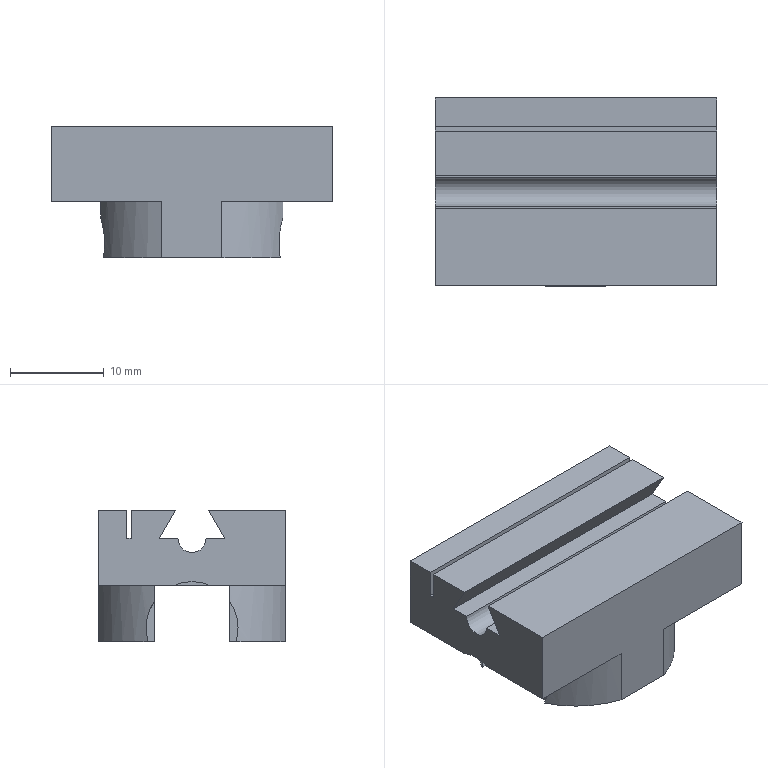Component | SolidWorks | Slider3-3 | 1 solid | 48 faces | volume 4822 mm3 | plane 27 | cylinder 21 | commonest cylinder face diameters 9.8 x8 2 x6 21 x4 15 x2 3 x1